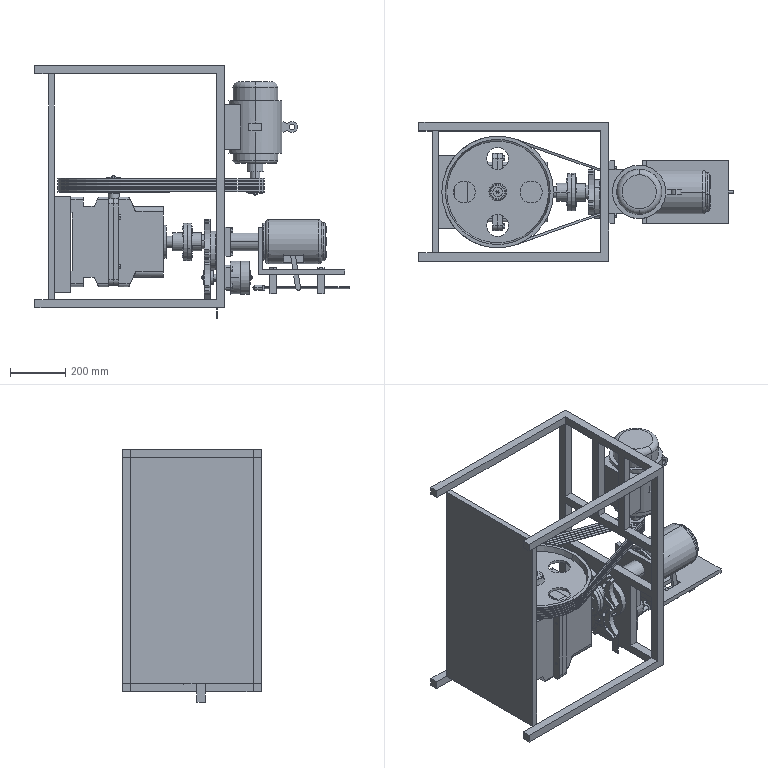Assembly | SolidWorks | mm | 45 component files | 46 solids | 1684 faces | box 1140.79 x 504 x 918.01 mm | volume 50447979 mm3 | plane 1056 | cylinder 428 | cone 120 | torus 64 | spline 16 | commonest cylinder face diameters 12 x36 40 x36 50 x30 20 x28 35 x24 64 x24 8 x20 48 x20
Bill of materials:
AxisOne | 1 |  | Solid stepped cylindrical shaft with about seven coaxial diameter sections; the largest section is near the middle and the diameters get smaller toward one end, with a short smaller pilot section at the other end.
AxisThree | 1 |  | Solid stepped cylindrical shaft or pin with five diameter sections that get larger toward one end. The smallest end is chamfered and the largest end is a flat face.
AxisTwo | 1 |  | Solid stepped cylindrical shaft with a raised narrow collar near the middle and a stepped-down journal on each side.
Bearing_2 | 2 |  | Thin flat annular ring (washer-like) with a large central through hole relative to its outer diameter, and a slight edge break at the bore.
Bearing | 1 |  | Annular ring like the previous ring part, but with a smaller central bore relative to the outer diameter and a slightly greater thickness.
BearingNew | 2 |  | Thick annular ring or spacer-like bushing with a central through bore and flat parallel end faces.
Belt | 5 |  | Very thin closed-loop band or flat strip outline in a teardrop shape: a large rounded end joined by two straight tangent sides to a small rounded end.
BevelGear | 1 |  | Toothed disc with a conical toothed face, like a straight-tooth bevel gear. The top face has a shallow dished recess, and a short hollow cylindrical hub with a through bore sits at its center. The rectangular teeth run down a conical frustum that narrows away from the top face.
BevelGear | 1 |  | Bevel-gear-like toothed disc. Many straight teeth are arranged on a conical face, the back face is recessed, and a cylindrical hub on the back has a central through bore.
Boss | 1 |  | Simple solid rectangular block or plate with flat faces and sharp edges.
Box | 1 |  | Machined-block or bracket-like housing half with a rectangular body. It has an open central pocket or cavity, two semicircular cutouts on opposite ends that line up on a common axis, a rounded-corner flange plate with four small holes near its corners, and a longitudinal slot or channel along the opposite side.
BoxCover | 1 |  | Block-shaped housing with a rounded-corner flange plate on one side and a rectangular main body. A raised circular boss with a central through bore sits on the face opposite the flange. A semicircular cutout and a narrow transverse groove are visible in the side profile, and small protrusions sit on the flange edge.
CamAxis | 1 |  | Long stepped cylindrical shaft with a larger-diameter cylindrical section near one end. That section carries a single helical ridge or groove, like a worm or screw thread, and is followed by a smaller end journal.
CamMachineCasing | 1 |  | Hollow cylindrical sleeve/tube with a concentric through bore and rounded (filleted) outer end edges.
Coupling | 2 |  | Flanged bushing: a thin circular flange with a smaller cylindrical boss on one side and a central through hole.
FixedPlate | 1 |  | Rectangular base plate with rounded corners and a large cylindrical boss with a central bore. The boss has two smaller offset holes of different sizes, and there are small protrusions near the plate corners.
Frame | 1 |  | Open frame made of thin square bars. One end is a rectangular grid of vertical and horizontal members, with longitudinal bars running back from it to give U-shaped side profiles. The lower bay holds a plate with two round holes and a small downward tab.
GrooveWheel | 2 |  | Flat four-armed star-shaped plate with concave curved edges between the arms, a central round through hole, a radial slot along each arm, and a short cylindrical boss on one face.
LowerEndCap | 1 |  | Flanged washer/bushing: a thin flange disc with a rounded outer edge, a shorter, smaller-diameter hub on one side, and a central through hole with a stepped or recessed face.
Motor | 1 |  | Cylindrical housing with a domed end cap, a wider central band, a rectangular box on one side, a lug with a hole on the opposite side, and a stepped cylindrical shaft sticking out of the other end. Overall it looks like a simplified electric motor.
Part1 | 1 |  | Flat circular disc with one off-center through hole and a small cylindrical pin projecting from one face near the edge.
Part2 | 1 |  | L-shaped flat bar: a long arm with a rounded end and a short perpendicular arm with a transverse hole. Two cylindrical pins of different diameters project from the long arm.
Pulley | 1 |  | Multi-groove pulley-like disc: a rim with several parallel V-shaped grooves, a recessed web with a raised outer lip, four large circular lightening holes, and a small central hub with a bore.
RetainingRing,Gasket,Bolt | 5 |  | Thin flat circular disc with a central hexagonal boss on one face and a small cylindrical pin on top of the hexagon.
RockerArm | 1 |  | Long slender cylindrical rod fixed perpendicular to a short rectangular crossbar. The crossbar carries two pointed-tip cylindrical pins of different diameters, one at each end, projecting the opposite way from the rod.
RotatingDisk | 1 |  | Thick circular disc with one large central through-bore and four smaller through-holes spaced evenly around it, like a flange.
Sleeve | 1 |  | Short ring with a thin wall: a hollow cylinder whose bore is large compared with its outer diameter.
SmallPulley | 1 |  | Hollow cylinder with a central through-bore and a stack of about six equally spaced outer ribs or flanges with tapered faces and smaller-diameter grooves between them.
SmallThrustBearing | 1 |  | Bushing or spacer with a thick wall: a short hollow cylinder with a central through-bore and a small chamfer or step at the bore edge.
SupportPlate | 1 |  | Thin flat rectangular plate with no visible holes or features.
SupportPlate2 | 1 |  | L-shaped bracket. An upright plate with a large round through-hole meets a flat base plate that has a rectangular cutout. Two small multi-faceted pegs pass through the base, sticking out a little above it and further below it.
SupportPlate3 | 1 |  | Rectangular mounting plate with a hollow cylindrical tube standing out from the middle of one face, and four small faceted stubs near the corners of the same face.
UpperEndCap | 1 |  | Circular disc or cap with rounded rim edges. A shorter cylindrical boss of smaller diameter is on one face, and six small rectangular tabs or pins are spaced around a circle on the opposite face.
Mates:
1. coincident | SupportPlate-1 face at (-180.267, 237.31, -320) dir (0, 0, -1) | Frame-1 face at (409.733, 267.31, -320) dir (0, 0, 1)
2. coincident | SupportPlate-1 face at (-180.267, -206.69, -320) dir (0, -1, 0) | Frame-1 face at (-250.267, -206.69, 90) dir (0, 1, 0)
3. distance | SupportPlate-1 face at (-200.267, 15.31, 90) dir (-1, 0, 0) | Frame-1 face at (-250.267, -236.69, -350) dir (-1, 0, 0)
4. distance | Boss-1 face at (-120.267, -115.69, -295) dir (0, -1, 0) | Frame-1 face at (-250.267, -206.69, 90) dir (0, 1, 0)
5. coincident | SupportPlate-1 face at (-180.267, 15.31, 90) dir (1, 0, 0) | Boss-1 face at (-180.267, 15.31, -120) dir (-1, 0, 0)
6. distance | Boss-1 face at (-120.267, 146.31, -295) dir (0, 0, -1) | SupportPlate-1 face at (-180.267, 237.31, -320) dir (0, 0, -1)
7. coincident | Box-1 face at (-120.267, 113.31, -262.5) dir (-1, 0, 0) | Boss-1 face at (-120.267, 15.31, -120) dir (1, 0, 0)
8. parallel | Box-1 face at (-120.267, -92.69, 42.5) dir (0, -1, 0) | Boss-1 face at (-120.267, -115.69, -295) dir (0, -1, 0)
9. distance | Box-1 face at (-120.267, -92.69, 42.5) dir (0, -1, 0) | Boss-1 face at (-120.267, -115.69, -295) dir (0, -1, 0)
10. distance | Box-1 face at (-120.267, 113.31, -272.5) dir (0, 0, -1) | Boss-1 face at (-120.267, 146.31, -295) dir (0, 0, -1)
11. concentric | Box-1 face at (35.733, 15.31, -452.5) dir (0, 0, 1) r 50 | BearingNew-1 face at (35.733, 15.31, 24.5) dir (0, 0, -1) r 45
12. coincident | Box-1 face at (-105.267, 91.31, -0.5001) dir (0, 0, -1) | BearingNew-1 face at (35.733, 15.31, -0.5001) dir (0, 0, -1)
13. concentric | Box-1 face at (35.733, 15.31, -452.5) dir (0, 0, 1) r 50 | BearingNew-2 face at (35.733, 15.31, -219.5) dir (0, 0, -1) r 45
14. coincident | Box-1 face at (-105.267, 91.31, -219.5) dir (0, 0, 1) | BearingNew-2 face at (35.733, 15.31, -219.5) dir (0, 0, 1)
15. coincident | AxisOne-1 edge at (35.733, 15.31, -244.5) dir (0, 0, -1) r 22.5 | BearingNew-2 face at (35.733, 15.31, -244.5) dir (0, 0, -1)
16. concentric | AxisOne-1 face at (35.733, 15.31, -246.5) dir (0, 0, -1) r 27.5 | BearingNew-2 face at (35.733, 15.31, -219.5) dir (0, 0, -1) r 22.5
17. coincident | AxisOne-1 face at (35.733, 15.31, 121.5) dir (0, 0, 1) | RetainingRing,Gasket,Bolt-1 face at (35.733, 15.31, 121.5) dir (0, 0, -1)
18. concentric | AxisOne-1 edge at (35.733, 15.31, 121.5) dir (0, 0, -1) r 17.5 | RetainingRing,Gasket,Bolt-1 edge at (35.733, 15.31, 124.5) dir (0, 0, 1) r 25
19. concentric | AxisOne-1 face at (35.733, 15.31, -246.5) dir (0, 0, -1) r 17.5 | Pulley-1 face at (35.733, 15.31, 69.5) dir (0, 0, -1) r 17.5
20. coincident | RetainingRing,Gasket,Bolt-1 face at (35.733, 15.31, 121.5) dir (0, 0, -1) | Pulley-1 face at (35.733, 218.31, 121.5) dir (0, 0, 1)
21. coincident | Frame-1 face at (439.733, 252.31, 90) dir (1, 0, 0) | Motor-1 face at (439.733, 15.31, 211.072) dir (-1, 0, 0)
22. coincident | Frame-1 face at (409.733, -64.69, 90) dir (0, -1, 0) | Motor-1 face at (504.733, -64.69, 226.072) dir (0, -1, 0)
23. concentric | Motor-1 face at (549.733, 15.31, 100.072) dir (0, 0, 1) r 17.5 | SmallPulley-1 face at (549.733, 15.31, 121.5) dir (0, 0, 1) r 17.5
24. coincident | Pulley-1 face at (35.733, 218.31, 69.5) dir (0, 0, -1) | SmallPulley-1 face at (549.733, 47.31, 69.5) dir (0, 0, -1)
25. coincident | SmallPulley-1 face at (549.733, 47.31, 69.5) dir (0, 0, -1) | RetainingRing,Gasket,Bolt-3 face at (549.733, 15.31, 69.5) dir (0, 0, 1)
26. concentric | SmallPulley-1 face at (549.733, 15.31, 121.5) dir (0, 0, 1) r 17.5 | RetainingRing,Gasket,Bolt-3 edge at (549.733, 15.31, 66.5) dir (0, 0, -1) r 25
27. coincident | Box-1 face at (17.733, -124.69, 27.5) dir (0, -1, 0) | BoxCover-1 face at (53.733, -124.69, -247.5) dir (0, -1, 0)
28. coincident | Box-1 face at (17.733, 135.31, -267.5) dir (0, 0, -1) | BoxCover-1 face at (53.733, 135.31, -267.5) dir (0, 0, -1)
29. concentric | BearingNew-2 edge at (35.733, 15.31, -244.5) dir (0, 0, 1) r 45 | BoxCover-1 face at (35.733, 15.31, 232.5) dir (0, 0, -1) r 50
30. lock | Frame-1 reference at (0, 0, 0) dir (1, 0, 0) | Motor-1 reference at (0, 0, 0) dir (1, 0, 0)
31. distance | Belt-1 face at (35.733, 15.31, 118.482) dir (0, 0, 1) | SmallPulley-1 face at (549.733, 47.31, 121.5) dir (0, 0, 1)
32. concentric | SmallPulley-1 edge at (549.733, 15.31, 108.499) dir (0, 0, 1) r 32 | Belt-2 face at (549.733, 15.31, 101.982) dir (0, 0, 1) r 24
33. distance | Belt-2 face at (35.733, 15.31, 108.482) dir (0, 0, 1) | Belt-1 face at (35.733, 15.31, 111.982) dir (0, 0, -1)
34. concentric | SmallPulley-1 edge at (549.733, 15.31, 98.499) dir (0, 0, 1) r 32 | Belt-3 face at (549.733, 15.31, 91.982) dir (0, 0, 1) r 24
35. distance | Belt-3 face at (35.733, 15.31, 98.482) dir (0, 0, 1) | Belt-2 face at (35.733, 15.31, 101.982) dir (0, 0, -1)
36. concentric | SmallPulley-1 edge at (549.733, 15.31, 88.499) dir (0, 0, 1) r 32 | Belt-5 face at (549.733, 15.31, 81.982) dir (0, 0, 1) r 24
37. distance | Belt-5 face at (35.733, 15.31, 88.482) dir (0, 0, 1) | Belt-3 face at (35.733, 15.31, 91.982) dir (0, 0, -1)
38. concentric | SmallPulley-1 edge at (549.733, 15.31, 78.499) dir (0, 0, 1) r 32 | Belt-4 face at (549.733, 15.31, 71.982) dir (0, 0, 1) r 24
39. distance | Belt-4 face at (35.733, 15.31, 78.482) dir (0, 0, 1) | Belt-5 face at (35.733, 15.31, 81.982) dir (0, 0, -1)
40. coincident | Belt-1 face at (560.379, -14.867, 111.982) dir (0.3327, -0.943, 0) | Belt-2 face at (560.379, -14.867, 101.982) dir (0.3327, -0.943, 0)
41. coincident | Belt-2 face at (560.379, -14.867, 101.982) dir (0.3327, -0.943, 0) | Belt-3 face at (560.379, -14.867, 91.982) dir (0.3327, -0.943, 0)
42. coincident | Belt-3 face at (560.379, -14.867, 91.982) dir (0.3327, -0.943, 0) | Belt-5 face at (560.379, -14.867, 81.982) dir (0.3327, -0.943, 0)
43. coincident | Belt-4 face at (560.379, -14.867, 71.982) dir (0.3327, -0.943, 0) | Belt-5 face at (560.379, -14.867, 81.982) dir (0.3327, -0.943, 0)
44. coincident | BoxCover-1 face at (178.528, 15.31, -110) dir (1, 0, 0) | Bearing-1 face at (178.528, 15.31, -110) dir (-1, 0, 0)
45. concentric | BoxCover-1 edge at (226.528, 15.31, -110) dir (1, 0, 0) r 45 | Bearing-1 edge at (200.528, 15.31, -110) dir (1, 0, 0) r 45
46. coincident | AxisTwo-1 face at (200.528, 40.31, -110) dir (-1, 0, 0) | Bearing-1 face at (200.528, 15.31, -110) dir (1, 0, 0)
47. concentric | BoxCover-1 face at (35.733, 15.31, -110) dir (1, 0, 0) r 45 | AxisTwo-1 face at (100.528, 15.31, -110) dir (-1, 0, 0) r 17.5
48. coincident | Coupling-1 face at (302.528, 15.31, -110) dir (1, 0, 0) | Coupling-2 face at (302.528, 15.31, -110) dir (-1, 0, 0)
49. concentric | Coupling-1 face at (302.528, 15.31, -110) dir (-1, 0, 0) r 68 | Coupling-2 face at (302.528, 15.31, -110) dir (1, 0, 0) r 68
50. coincident | AxisTwo-1 face at (250.528, 33.81, -110) dir (1, 0, 0) | Coupling-1 face at (250.528, 15.31, -110) dir (-1, 0, 0)
51. concentric | AxisTwo-1 face at (100.528, 15.31, -110) dir (-1, 0, 0) r 17.5 | Coupling-1 face at (288.528, 15.31, -110) dir (-1, 0, 0) r 33
52. coincident | AxisTwo-1 face at (150.528, 35.31, -110) dir (-1, 0, 0) | BevelGear-2 face at (150.528, 15.31, -110) dir (1, 0, 0)
53. concentric | AxisTwo-1 face at (100.528, 15.31, -110) dir (-1, 0, 0) r 17.5 | BevelGear-2 edge at (139.4, 15.31, -110) dir (1, 0, 0) r 77.151
54. coincident | BevelGear-2 face at (99.528, 15.31, -110) dir (-1, 0, 0) | RetainingRing,Gasket,Bolt-4 face at (99.528, 15.31, -110) dir (1, 0, 0)
55. concentric | BevelGear-2 face at (150.528, 15.31, -110) dir (1, 0, 0) r 28 | RetainingRing,Gasket,Bolt-4 face at (96.528, 15.31, -110) dir (1, 0, 0) r 25
56. coincident | Coupling-2 face at (354.528, 15.31, -110) dir (1, 0, 0) | CamAxis-1 face at (354.528, 32.948, -104.418) dir (-1, 0, 0)
57. concentric | Coupling-2 face at (316.528, 15.31, -110) dir (1, 0, 0) r 33 | CamAxis-1 face at (789.528, 15.31, -110) dir (1, 0, 0) r 22.5
58. coincident | Coupling-2 face at (354.528, 15.31, -110) dir (1, 0, 0) | GrooveWheel-1 face at (354.528, 15.31, -110) dir (-1, 0, 0)
59. concentric | Coupling-2 face at (316.528, 15.31, -110) dir (1, 0, 0) r 33 | GrooveWheel-1 face at (354.528, 15.31, -110) dir (1, 0, 0) r 25
60. concentric | CamAxis-1 face at (789.528, 15.31, -110) dir (1, 0, 0) r 22.5 | Part1-1 face at (405.528, 15.31, -110) dir (-1, 0, 0) r 20
61. coincident | GrooveWheel-1 face at (385.528, 15.31, -110) dir (1, 0, 0) | Part1-1 face at (385.528, -9.187, -141.621) dir (-1, 0, 0)
62. coincident | Frame-1 face at (439.733, 252.31, 90) dir (1, 0, 0) | SupportPlate3-1 face at (439.733, 15.31, -110) dir (-1, 0, 0)
63. concentric | CamAxis-1 face at (789.528, 15.31, -110) dir (1, 0, 0) r 22.5 | SupportPlate3-1 face at (459.733, 15.31, -110) dir (1, 0, 0) r 33
64. parallel | Frame-1 face at (58.516, -97.69, -52) dir (0, -1, 0) | SupportPlate3-1 face at (439.733, -98.19, -163) dir (0, -1, 0)
65. coincident | Frame-1 face at (58.516, -97.69, -52) dir (0, -1, 0) | SupportPlate2-1 face at (577.733, -97.69, 0.9999) dir (0, -1, 0)
66. concentric | CamAxis-1 face at (789.528, 15.31, -110) dir (1, 0, 0) r 25 | LowerEndCap-1 face at (587.733, 15.31, -110) dir (1, 0, 0) r 44.5
67. concentric | LowerEndCap-1 face at (587.733, 15.31, -110) dir (1, 0, 0) r 44.5 | Bearing_2-1 face at (619.523, 15.31, -110) dir (-1, 0, 0) r 45
68. coincident | LowerEndCap-1 face at (602.733, 15.31, -110) dir (1, 0, 0) | Bearing_2-1 face at (602.733, 15.31, -110) dir (-1, 0, 0)
69. concentric | CamAxis-1 face at (789.528, 15.31, -110) dir (1, 0, 0) r 25 | CamMachineCasing-1 face at (587.733, 15.31, -110) dir (-1, 0, 0) r 56
70. coincident | LowerEndCap-1 face at (587.733, 15.31, -110) dir (1, 0, 0) | CamMachineCasing-1 face at (587.733, 15.31, -110) dir (-1, 0, 0)
71. coincident | CamAxis-1 face at (739.528, 55.829, -97.177) dir (1, 0, 0) | Sleeve-1 face at (739.528, 15.31, -110) dir (-1, 0, 0)
72. concentric | CamAxis-1 face at (789.528, 15.31, -110) dir (1, 0, 0) r 25 | Sleeve-1 face at (759.528, 15.31, -110) dir (-1, 0, 0) r 25
73. concentric | CamAxis-1 face at (789.528, 15.31, -110) dir (1, 0, 0) r 25 | Bearing_2-2 face at (776.318, 15.31, -110) dir (-1, 0, 0) r 25
74. coincident | Sleeve-1 face at (759.528, 15.31, -110) dir (1, 0, 0) | Bearing_2-2 face at (759.528, 15.31, -110) dir (-1, 0, 0)
75. coincident | UpperEndCap-1 face at (790.733, 15.31, -110) dir (-1, 0, 0) | CamMachineCasing-1 face at (790.733, 15.31, -110) dir (1, 0, 0)
76. concentric | UpperEndCap-1 face at (790.733, 15.31, -110) dir (-1, 0, 0) r 69.5 | CamMachineCasing-1 face at (587.733, 15.31, -110) dir (-1, 0, 0) r 80
77. concentric | SupportPlate2-1 edge at (800.233, 15.81, -277) dir (1, 0, 0) r 5 | RockerArm-1 face at (584.528, 15.81, -277) dir (1, 0, 0) r 4
78. concentric | Frame-1 face at (-250.267, 15.31, -240) dir (1, 0, 0) r 17.5 | AxisThree-1 face at (365.528, 15.31, -240) dir (-1, 0, 0) r 22
79. coincident | GrooveWheel-1 face at (365.528, 15.31, -110) dir (-1, 0, 0) | AxisThree-1 face at (365.528, 18.139, -246.403) dir (-1, 0, 0)
80. concentric | AxisThree-1 face at (365.528, 15.31, -240) dir (-1, 0, 0) r 10 | GrooveWheel-2 face at (396.528, 15.31, -240) dir (-1, 0, 0) r 25
81. coincident | GrooveWheel-1 face at (365.528, 15.31, -110) dir (-1, 0, 0) | GrooveWheel-2 face at (365.528, 15.31, -240) dir (-1, 0, 0)
82. coincident | GrooveWheel-2 face at (365.528, 15.31, -240) dir (-1, 0, 0) | RetainingRing,Gasket,Bolt-5 face at (365.528, 15.31, -240) dir (1, 0, 0)
83. concentric | GrooveWheel-2 face at (396.528, 15.31, -240) dir (-1, 0, 0) r 20 | RetainingRing,Gasket,Bolt-5 face at (362.528, 15.31, -240) dir (1, 0, 0) r 25
84. concentric | AxisThree-1 face at (365.528, 15.31, -240) dir (-1, 0, 0) r 22 | FixedPlate-1 face at (459.733, 15.31, -240) dir (1, 0, 0) r 34
85. parallel | Frame-1 face at (58.516, -97.69, -52) dir (0, -1, 0) | FixedPlate-1 face at (459.733, -85.19, -275) dir (0, -1, 0)
86. coincident | Frame-1 face at (439.733, 252.31, 90) dir (1, 0, 0) | FixedPlate-1 face at (439.733, -75.19, -275) dir (-1, 0, 0)
87. concentric | AxisThree-1 face at (365.528, 15.31, -240) dir (-1, 0, 0) r 22 | RetainingRing,Gasket,Bolt-6 edge at (528.528, 15.31, -240) dir (1, 0, 0) r 25
88. coincident | AxisThree-1 face at (528.528, 15.31, -240) dir (1, 0, 0) | RetainingRing,Gasket,Bolt-6 face at (528.528, 15.31, -240) dir (-1, 0, 0)
89. concentric | AxisThree-1 face at (365.528, 15.31, -240) dir (-1, 0, 0) r 22 | SmallThrustBearing-1 face at (489.523, 15.31, -240) dir (-1, 0, 0) r 34
90. coincident | FixedPlate-1 edge at (459.733, 15.31, -240) dir (1, 0, 0) r 34 | SmallThrustBearing-1 face at (459.733, 15.31, -240) dir (-1, 0, 0)
91. coincident | RetainingRing,Gasket,Bolt-6 face at (528.528, 15.31, -240) dir (-1, 0, 0) | RotatingDisk-1 face at (528.528, 15.31, -240) dir (1, 0, 0)
92. concentric | AxisThree-1 face at (365.528, 15.31, -240) dir (-1, 0, 0) r 22 | RotatingDisk-1 face at (528.528, 15.31, -240) dir (-1, 0, 0) r 22
93. coincident | SupportPlate2-1 face at (577.733, -97.69, -57) dir (0, 0, 1) | SupportPlate3-1 face at (439.733, 128.81, -57) dir (0, 0, 1)
94. distance | RockerArm-1 face at (576.528, 15.81, -277) dir (-1, 0, 0) | RetainingRing,Gasket,Bolt-6 face at (528.528, 15.31, -240) dir (-1, 0, 0)
95. coincident | SupportPlate3-1 face at (577.733, 15.31, -110) dir (1, 0, 0) | LowerEndCap-1 face at (577.733, 15.31, -110) dir (-1, 0, 0)
96. parallel | Frame-1 face at (-250.267, -236.69, 90) dir (0, -1, 0) | CamMachineCasing-1 face at (652.828, -12.98, -70) dir (0, -1, 0)
97. concentric | CamMachineCasing-1 face at (689.233, 7.02, -172.831) dir (0, -1, 0) r 6 | Part2-1 face at (689.233, -22.052, -172.831) dir (0, -1, 0) r 6
98. lock | CamMachineCasing-1 reference at (0, 0, 0) dir (1, 0, 0) | Part2-1 reference at (0, 0, 0) dir (1, 0, 0)
99. coincident | SupportPlate2-1 face at (577.733, -97.69, -212) dir (1, 0, 0) | LowerEndCap-1 face at (577.733, 15.31, -110) dir (-1, 0, 0)
100. concentric | SmallPulley-1 edge at (549.733, 15.31, 118.499) dir (0, 0, 1) r 32 | Belt-1 face at (549.733, 15.31, 111.982) dir (0, 0, 1) r 24
101. lock | AxisOne-1 reference at (0, 0, 0) dir (1, 0, 0) | BevelGear-1 reference at (0, 0, 0) dir (1, 0, 0)